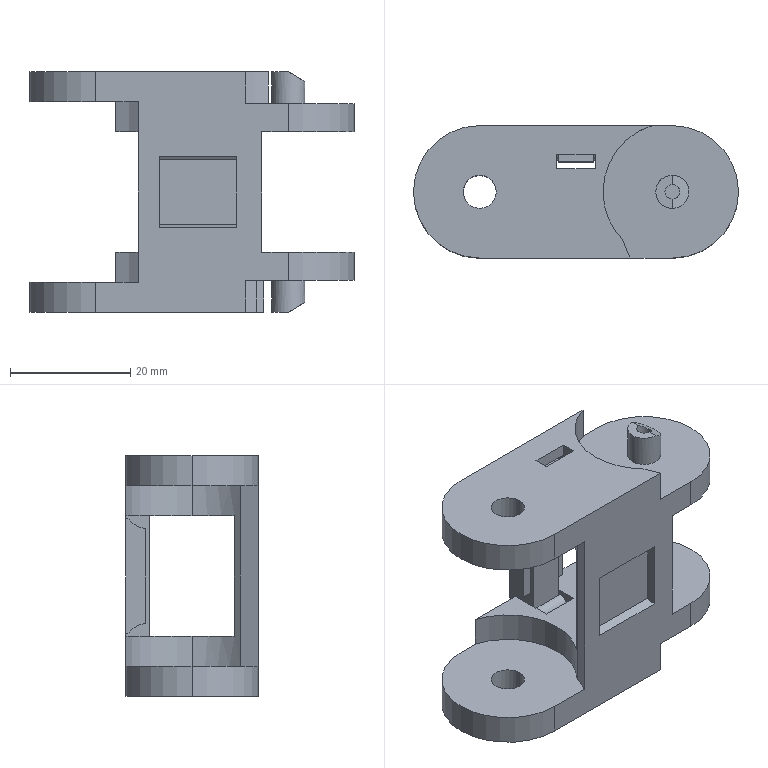Component | SolidWorks | MHPUS204-38-33-A-1_12-1 | 1 solid | 94 faces | volume 15041 mm3 | plane 51 | cylinder 43 | commonest cylinder face diameters 5.5 x8 22 x6 23 x6 3.4 x6 0.4 x6 2.444 x4 9.434 x4 4.8 x2